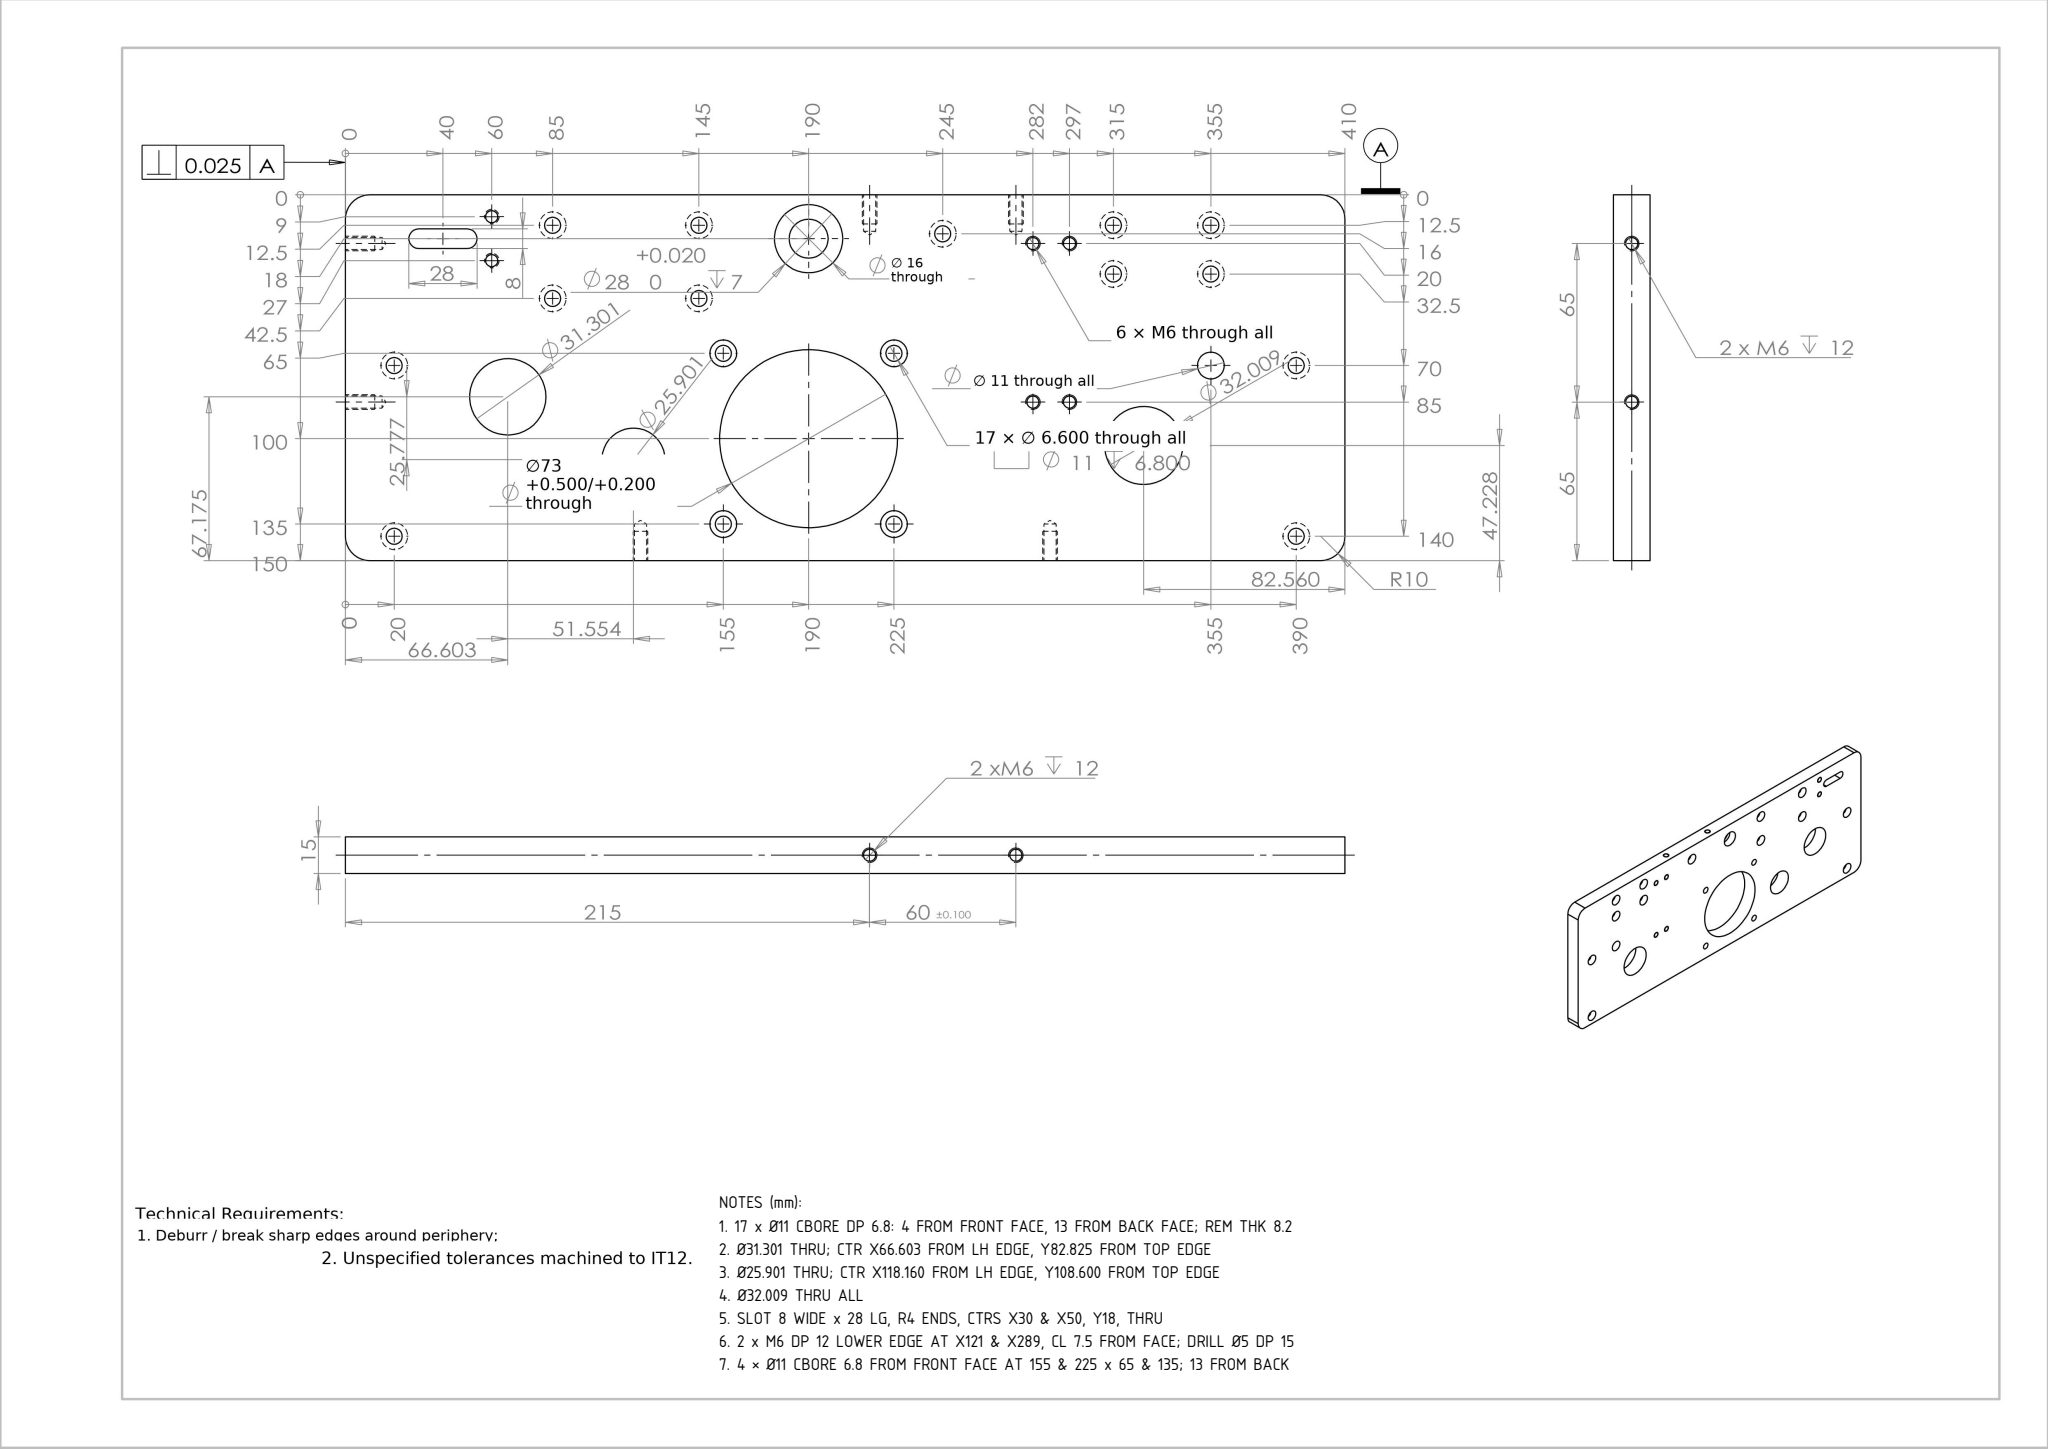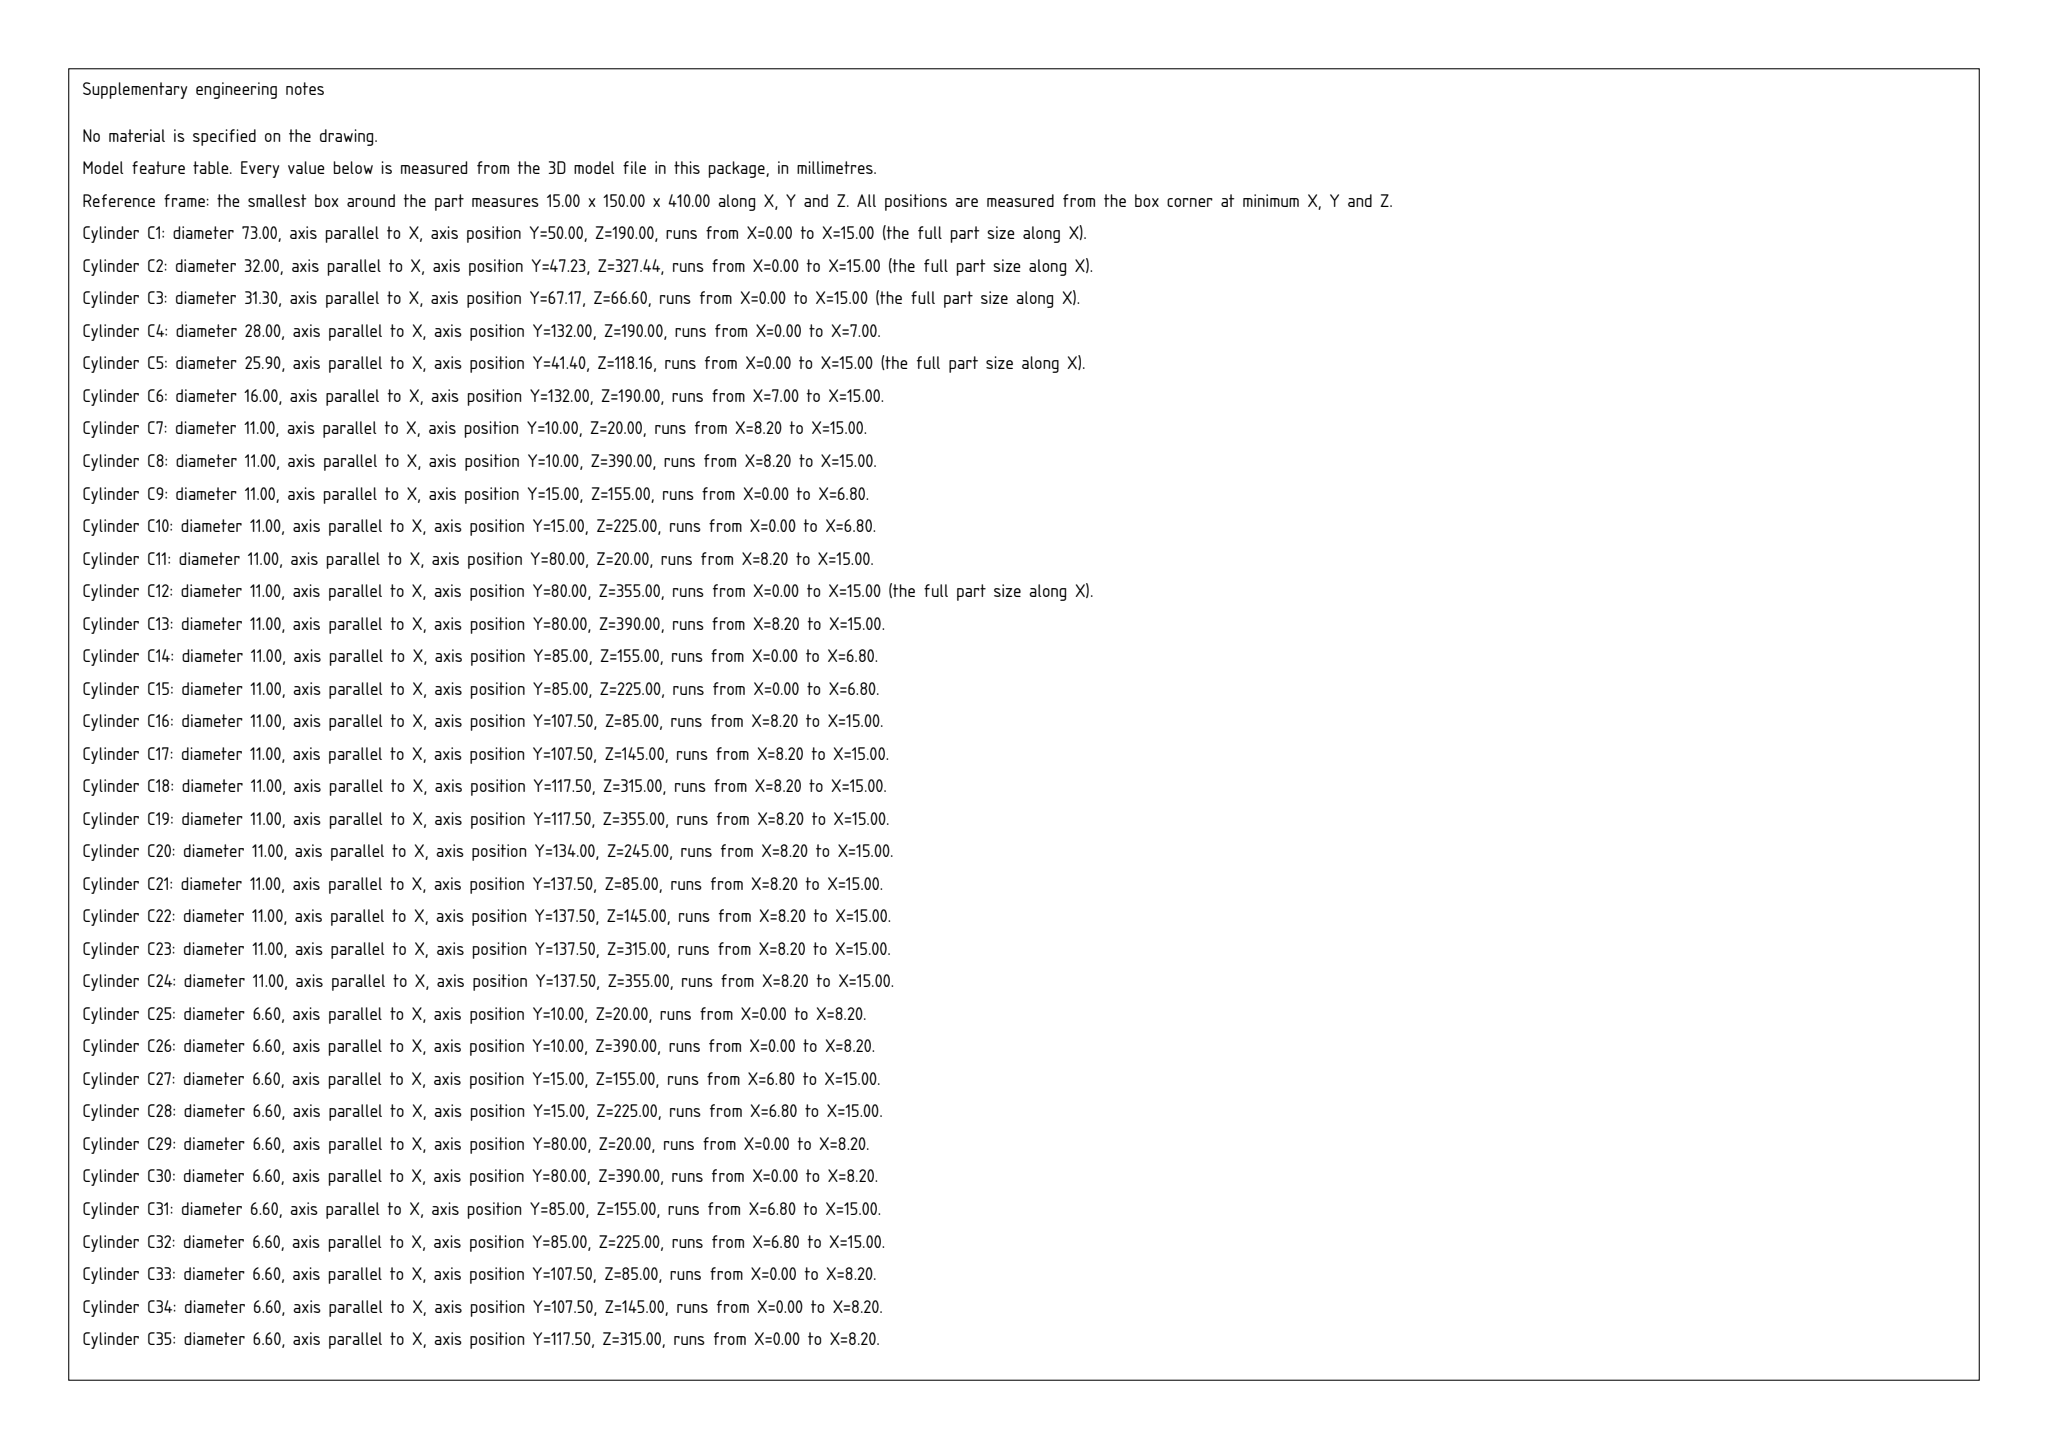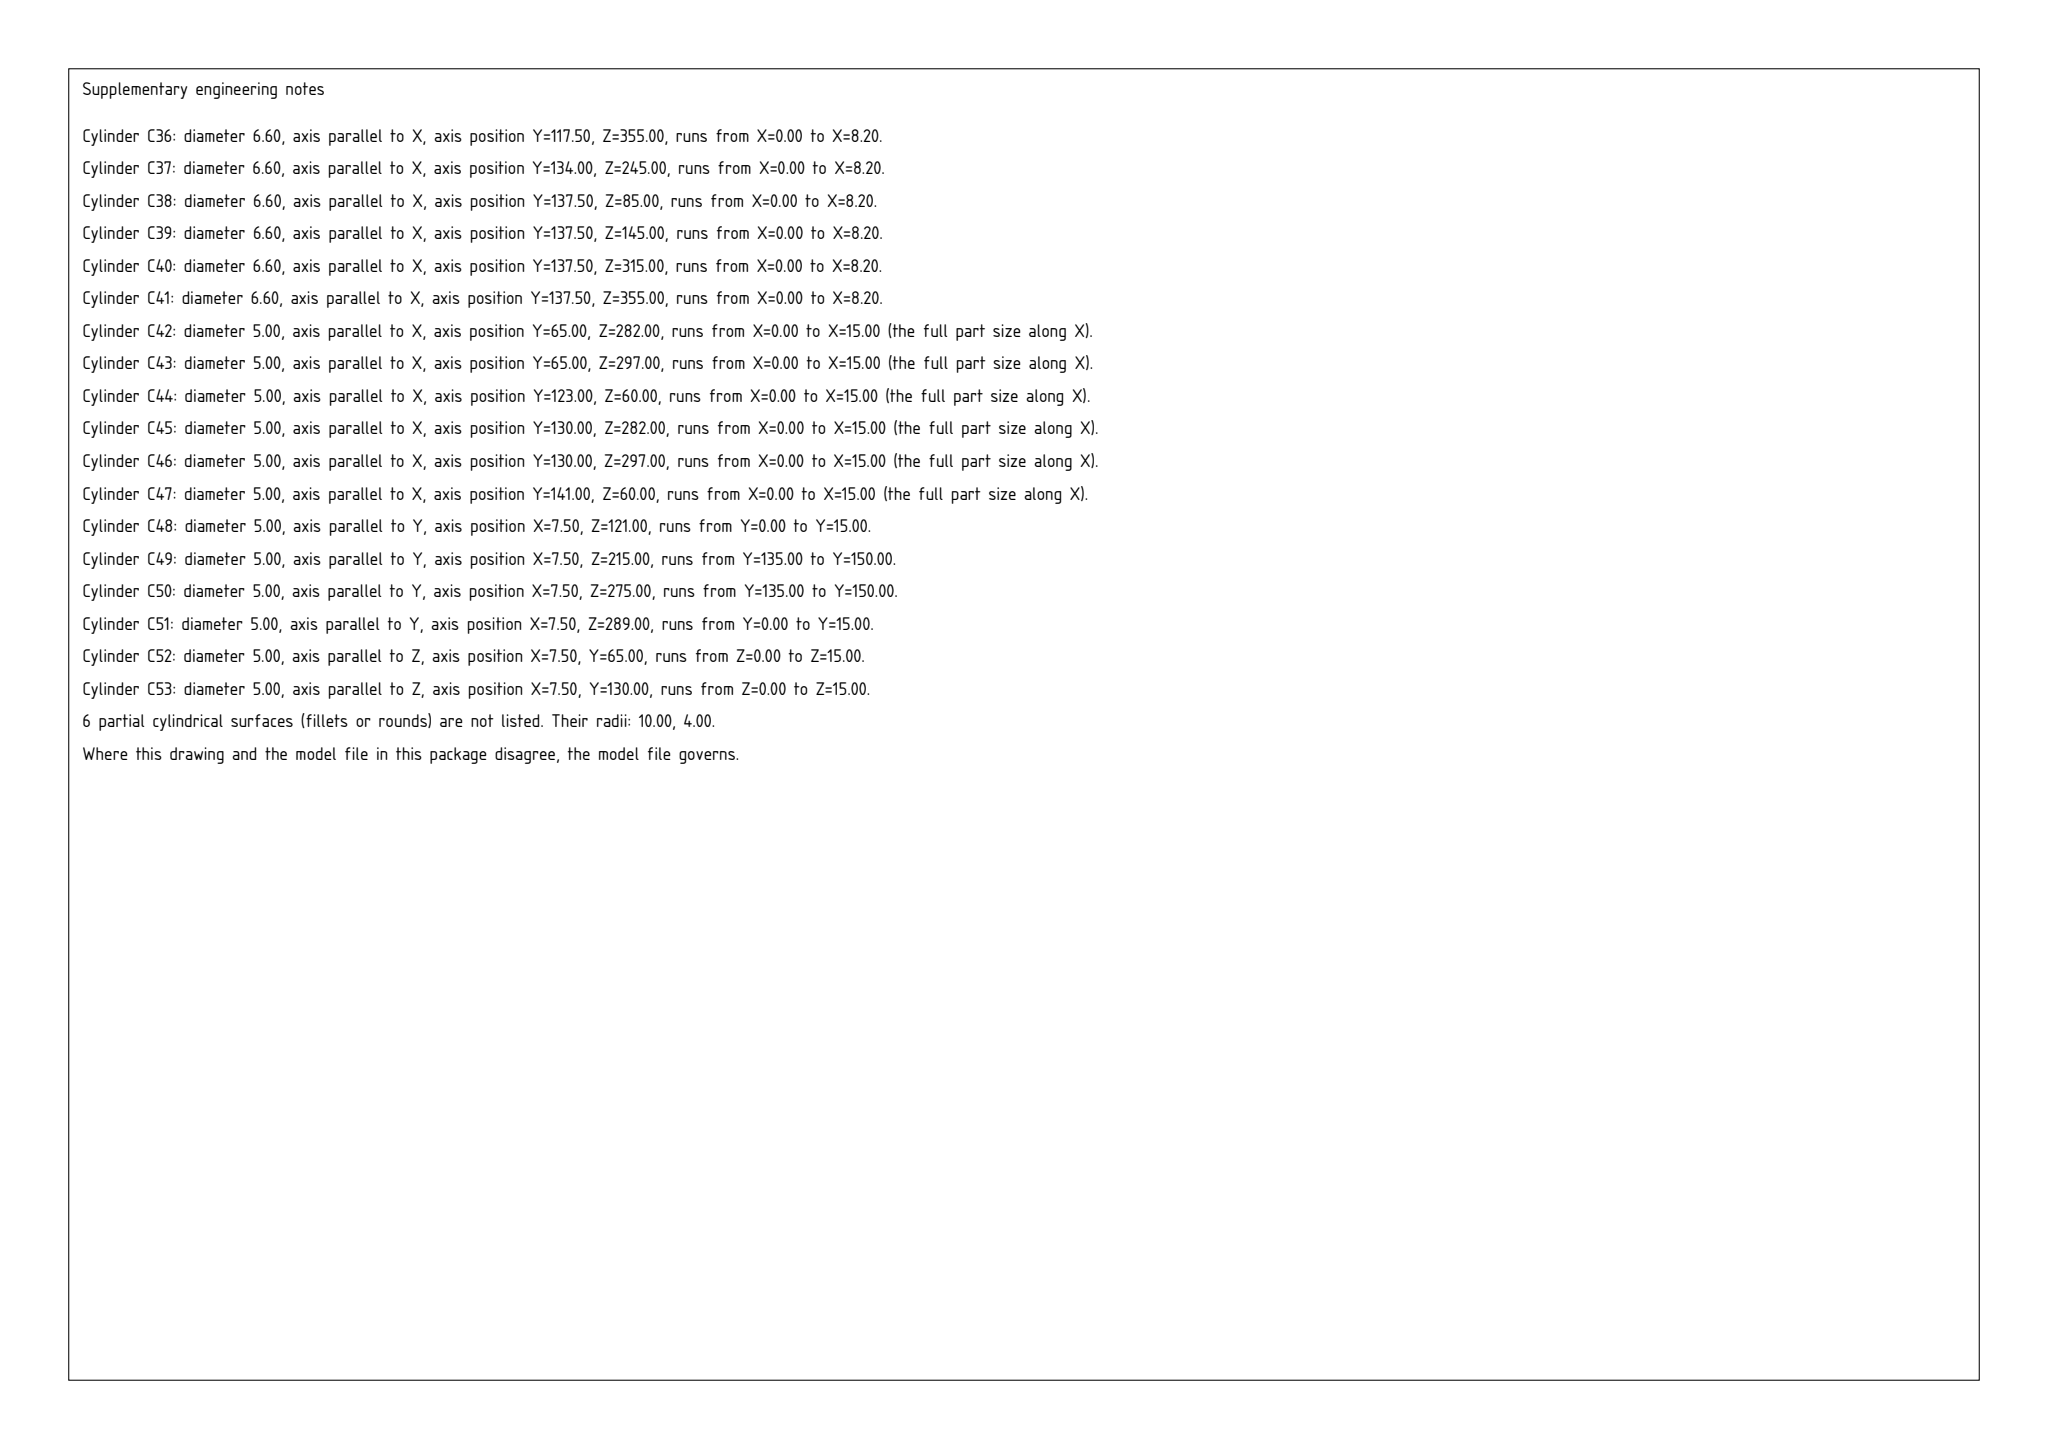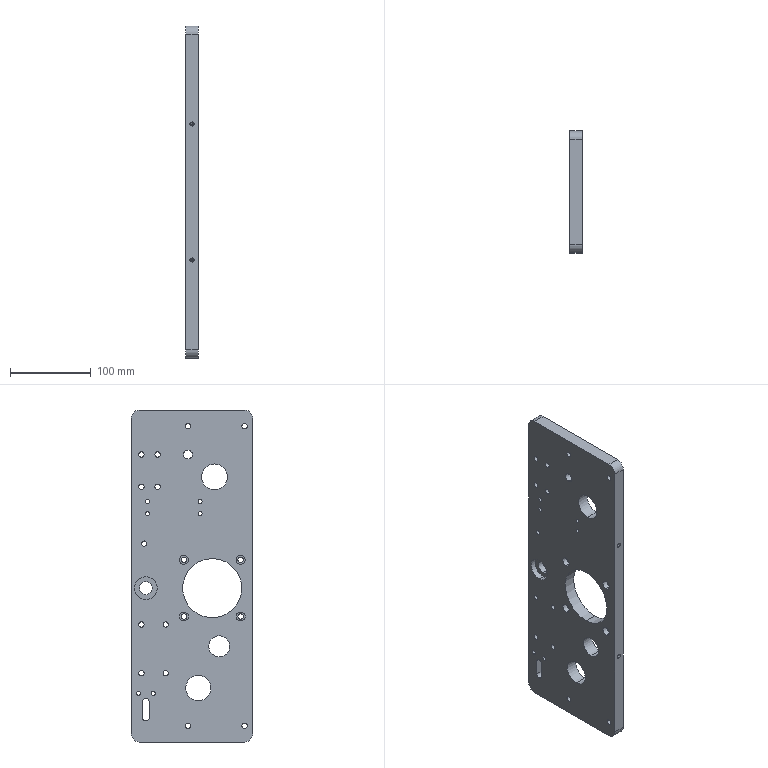Part | SolidWorks | mm | 1 solid | 151 faces | box 15 x 150 x 410 mm | volume 797070 mm3 | cylinder 113 | plane 26 | cone 12 | commonest cylinder face diameters 11 x36 6.6 x34 5 x24 20 x4 8 x3 32.009 x2 25.901 x2 31.301 x2
Drawing notes:
17 x Ø11 CBORE DP 6.8: 4 FROM FRONT FACE, 13 FROM BACK FACE; REM THK 8.2 | from the solid: axis_planes x=6.8 count 4 and x=8.2 count 13; Ø11 L6.8 x17 + Ø6.6 L8.2 x17 = 15 thk
Ø31.301 THRU; CTR X66.603 FROM LH EDGE, Y82.825 FROM TOP EDGE | from the solid: cyl Ø31.301 axis x at [y=67.17, z=66.6], L15 = plate thk; Y=150-67.175
Ø25.901 THRU; CTR X118.160 FROM LH EDGE, Y108.600 FROM TOP EDGE | from the solid: cyl Ø25.901 axis x at [y=41.4, z=118.16], L15 = plate thk; Y=150-41.4
Ø32.009 THRU ALL | from the solid: cyl Ø32.009 axis x at [y=47.23, z=327.44], L15 = plate thk
SLOT 8 WIDE x 28 LG, R4 ENDS, CTRS X30 & X50, Y18, THRU | from the solid: two Ø8 x-axis cyls at [y=132,z=30] and [y=132,z=50], L15 = thru; Y=150-132=18
2 x M6 DP 12 LOWER EDGE AT X121 & X289, CL 7.5 FROM FACE; DRILL Ø5 DP 15 | from the solid: Ø5 y-axis cyls at [x=7.5, z=121] and [x=7.5, z=289], L15; cone 118 deg ref dia 5
4 × Ø11 CBORE 6.8 FROM FRONT FACE AT 155 & 225 x 65 & 135; 13 FROM BACK | from the solid: axis_planes x=6.8 count 4 (c'bore floors opening at x=0 front face) vs x=8.2 count 13 (opening at x=15 back face); the 4 Ø11x6.8 c'bores grouped symmetric about Ø73 bore at y=15/85, z=155/225 -> 65/135 from top edge, 155/225 from left edge
build123d program:
from build123d import *

# Parameters (mm, degrees)
SKETCH1_W                                            = 360
SKETCH1_H                                            = 150
BOSS_EXTRUDE1_DEPTH                                  = 15
F_16_0_16_DIAMETER_HOLE2_D                           = 16
CUT_EXTRUDE1_DEPTH                                   = 391.288
M6_TAPPED_HOLE1_D                                    = 5
M6_TAPPED_HOLE1_DEPTH                                = 15
M6_TAPPED_HOLE1_TIP                                  = 1.502
HOLE_SIZE_ACCORDING_TO_HEX_SOCKET_HEAD_C_D           = 6.6
HOLE_SIZE_ACCORDING_TO_HEX_SOCKET_HEAD_C_CBORE_D     = 11
HOLE_SIZE_ACCORDING_TO_HEX_SOCKET_HEAD_C_CBORE_DEPTH = 6.8
HOLE_SIZE_ACCORDING_TO_HEX_SOCKET_HE_2_D             = 6.6
HOLE_SIZE_ACCORDING_TO_HEX_SOCKET_HE_2_CBORE_D       = 11
HOLE_SIZE_ACCORDING_TO_HEX_SOCKET_HE_2_CBORE_DEPTH   = 6.8
SKETCH27_R                                           = 14
CUT_EXTRUDE2_DEPTH                                   = 7
HOLE_SIZE_ACCORDING_TO_HEX_SOCKET_HE_3_D             = 6.6
HOLE_SIZE_ACCORDING_TO_HEX_SOCKET_HE_3_CBORE_D       = 11
HOLE_SIZE_ACCORDING_TO_HEX_SOCKET_HE_3_CBORE_DEPTH   = 6.8
M6_TAPPED_HOLE7_D                                    = 5
M6_TAPPED_HOLE7_DEPTH                                = 15
M6_TAPPED_HOLE7_TIP                                  = 1.502
SKETCH34_R                                           = 36.5
CUT_EXTRUDE5_DEPTH                                   = 391.288
HOLE_SIZE_ACCORDING_TO_HEX_SOCKET_HE_4_D             = 6.6
HOLE_SIZE_ACCORDING_TO_HEX_SOCKET_HE_4_CBORE_D       = 11
HOLE_SIZE_ACCORDING_TO_HEX_SOCKET_HE_4_CBORE_DEPTH   = 6.8
SKETCH39_W                                           = 15
SKETCH39_H                                           = 150
BOSS_EXTRUDE2_DEPTH                                  = 10
M6_TAPPED_HOLE6_D                                    = 5
M6_TAPPED_HOLE6_DEPTH                                = 15
M6_TAPPED_HOLE6_TIP                                  = 1.502
SKETCH40_W                                           = 15
SKETCH40_H                                           = 150
BOSS_EXTRUDE3_DEPTH                                  = 40
HOLE_SIZE_ACCORDING_TO_HEX_SOCKET_HE_5_D             = 6.6
HOLE_SIZE_ACCORDING_TO_HEX_SOCKET_HE_5_CBORE_D       = 11
HOLE_SIZE_ACCORDING_TO_HEX_SOCKET_HE_5_CBORE_DEPTH   = 6.8
M6_TAPPED_HOLE8_D                                    = 5
FILLET1_R                                            = 10
LPATTERN1_COUNT                                      = 2
LPATTERN1_PITCH                                      = 370
F_11_0_11_DIAMETER_HOLE1_D                           = 11
M6_TAPPED_HOLE9_D                                    = 5
M6_TAPPED_HOLE9_DEPTH                                = 15
M6_TAPPED_HOLE9_TIP                                  = 1.502
SKETCH49_R                                           = 16.004
SKETCH49_R_2                                         = 12.95
SKETCH49_R_3                                         = 15.65
CUT_EXTRUDE6_DEPTH                                   = 85


with BuildPart() as part:
    # Sketch1 → Boss-Extrude1 (new body)
    with BuildSketch(Plane(origin=(0, 0, 0), x_dir=(0, 0, -1), z_dir=(1, 0, 0))):
        with Locations((180, 75)):
            Rectangle(SKETCH1_W, SKETCH1_H)
    extrude(amount=BOSS_EXTRUDE1_DEPTH)

    # 16.0 _16_ Diameter Hole2 (through all)
    with Locations(Plane(origin=(15, 0, 0), x_dir=(0, 0, -1), z_dir=(1, 0, 0))):
        with Locations((180, 132)):
            Hole(F_16_0_16_DIAMETER_HOLE2_D / 2)

    # Sketch8 → Cut-Extrude1 (cut, through all)
    with BuildSketch(Plane(origin=(15, 0, 0), x_dir=(0, 0, -1), z_dir=(1, 0, 0))):
        with BuildLine():
            Line((320, 136), (340, 136))
            ThreePointArc((340, 136), (344, 132), (340, 128))
            Line((340, 128), (320, 128))
            ThreePointArc((320, 128), (316, 132), (320, 136))
        make_face()
    extrude(amount=-CUT_EXTRUDE1_DEPTH, mode=Mode.SUBTRACT)

    # M6 Tapped Hole1
    with Locations(Plane(origin=(15, 0, 0), x_dir=(0, 0, -1), z_dir=(1, 0, 0))):
        with Locations((310, 141), (310, 123)):
            Hole(M6_TAPPED_HOLE1_D / 2, depth=M6_TAPPED_HOLE1_DEPTH)
            with Locations((0, 0, -(M6_TAPPED_HOLE1_DEPTH + M6_TAPPED_HOLE1_TIP / 2))):  # 118° drill point
                Cone(0, M6_TAPPED_HOLE1_D / 2, M6_TAPPED_HOLE1_TIP, mode=Mode.SUBTRACT)

    # Hole Size according to Hex Socket Head C (through all)
    with Locations(Plane(origin=(15, 0, 0), x_dir=(0, 0, -1), z_dir=(1, 0, 0))):
        with Locations((350, 10), (350, 80)):
            hole_size_according_to_hex_socket_head_c = CounterBoreHole(HOLE_SIZE_ACCORDING_TO_HEX_SOCKET_HEAD_C_D / 2, HOLE_SIZE_ACCORDING_TO_HEX_SOCKET_HEAD_C_CBORE_D / 2, HOLE_SIZE_ACCORDING_TO_HEX_SOCKET_HEAD_C_CBORE_DEPTH)

    # Hole Size according to Hex Socket He 2 (through all)
    with Locations(Plane(origin=(15, 0, 0), x_dir=(0, 0, -1), z_dir=(1, 0, 0))):
        with Locations((285, 107.5), (225, 107.5), (285, 137.5), (225, 137.5)):
            CounterBoreHole(HOLE_SIZE_ACCORDING_TO_HEX_SOCKET_HE_2_D / 2, HOLE_SIZE_ACCORDING_TO_HEX_SOCKET_HE_2_CBORE_D / 2, HOLE_SIZE_ACCORDING_TO_HEX_SOCKET_HE_2_CBORE_DEPTH)

    # Sketch27 → Cut-Extrude2 (cut)
    with BuildSketch(Plane.ZY):
        with Locations((-180, 132)):
            Circle(SKETCH27_R)
    extrude(amount=-CUT_EXTRUDE2_DEPTH, mode=Mode.SUBTRACT)

    # Hole Size according to Hex Socket He 3 (through all)
    with Locations(Plane(origin=(15, 0, 0), x_dir=(0, 0, -1), z_dir=(1, 0, 0))):
        with Locations((125, 134)):
            CounterBoreHole(HOLE_SIZE_ACCORDING_TO_HEX_SOCKET_HE_3_D / 2, HOLE_SIZE_ACCORDING_TO_HEX_SOCKET_HE_3_CBORE_D / 2, HOLE_SIZE_ACCORDING_TO_HEX_SOCKET_HE_3_CBORE_DEPTH)

    # M6 Tapped Hole7
    with Locations(Plane(origin=(0, 150, 0), x_dir=(-1, 0, 0), z_dir=(0, 1, 0))):
        with Locations((-7.5, -155), (-7.5, -95)):
            Hole(M6_TAPPED_HOLE7_D / 2, depth=M6_TAPPED_HOLE7_DEPTH)
            with Locations((0, 0, -(M6_TAPPED_HOLE7_DEPTH + M6_TAPPED_HOLE7_TIP / 2))):  # 118° drill point
                Cone(0, M6_TAPPED_HOLE7_D / 2, M6_TAPPED_HOLE7_TIP, mode=Mode.SUBTRACT)

    # Sketch34 → Cut-Extrude5 (cut, through all)
    with BuildSketch(Plane.ZY):
        with Locations((-180, 50)):
            Circle(SKETCH34_R)
    extrude(amount=-CUT_EXTRUDE5_DEPTH, mode=Mode.SUBTRACT)

    # Hole Size according to Hex Socket He 4 (through all)
    with Locations(Plane.ZY):
        with Locations((-215, 85), (-145, 85), (-145, 15), (-215, 15)):
            CounterBoreHole(HOLE_SIZE_ACCORDING_TO_HEX_SOCKET_HE_4_D / 2, HOLE_SIZE_ACCORDING_TO_HEX_SOCKET_HE_4_CBORE_D / 2, HOLE_SIZE_ACCORDING_TO_HEX_SOCKET_HE_4_CBORE_DEPTH)

    # Sketch39 → Boss-Extrude2 (add)
    with BuildSketch(Plane(origin=(0, 0, -360), x_dir=(-1, 0, 0), z_dir=(0, 0, -1))):
        with Locations((-7.5, 75)):
            Rectangle(SKETCH39_W, SKETCH39_H)
    extrude(amount=BOSS_EXTRUDE2_DEPTH)

    # M6 Tapped Hole6
    with Locations(Plane(origin=(0.007088, 11.918, -370), x_dir=(-1, 0, 0), z_dir=(0, 0, -1))):
        with Locations((-7.493, 118.082), (-7.493, 53.082)):
            Hole(M6_TAPPED_HOLE6_D / 2, depth=M6_TAPPED_HOLE6_DEPTH)
            with Locations((0, 0, -(M6_TAPPED_HOLE6_DEPTH + M6_TAPPED_HOLE6_TIP / 2))):  # 118° drill point
                Cone(0, M6_TAPPED_HOLE6_D / 2, M6_TAPPED_HOLE6_TIP, mode=Mode.SUBTRACT)

    # Sketch40 → Boss-Extrude3 (add)
    with BuildSketch(Plane.XY):
        with Locations((7.5, 75)):
            Rectangle(SKETCH40_W, SKETCH40_H)
    extrude(amount=BOSS_EXTRUDE3_DEPTH)

    # Hole Size according to Hex Socket He 5 (through all)
    with Locations(Plane(origin=(15, 0, 0), x_dir=(0, 0, -1), z_dir=(1, 0, 0))):
        with Locations((15, 137.5), (55, 137.5), (55, 117.5), (15, 117.5)):
            CounterBoreHole(HOLE_SIZE_ACCORDING_TO_HEX_SOCKET_HE_5_D / 2, HOLE_SIZE_ACCORDING_TO_HEX_SOCKET_HE_5_CBORE_D / 2, HOLE_SIZE_ACCORDING_TO_HEX_SOCKET_HE_5_CBORE_DEPTH)

    # M6 Tapped Hole8 (through all)
    with Locations(Plane(origin=(15, 0, 0), x_dir=(0, 0, -1), z_dir=(1, 0, 0))):
        with Locations((73, 65), (73, 130), (88, 130), (88, 65)):
            Hole(M6_TAPPED_HOLE8_D / 2)

    # Fillet1
    fillet1_edges = [part.edges().sort_by_distance(p)[0] for p in [
        (7.5, 0, -370),
        (7.5, 150, -370),
        (7.5, 0, 40),
        (7.5, 150, 40),
    ]]
    fillet(fillet1_edges, radius=FILLET1_R)

    # LPattern1: Hole Size according to Hex Socket Head C ×2
    with Locations(*[(0, 0, i * LPATTERN1_PITCH) for i in range(1, LPATTERN1_COUNT)]):
        add(hole_size_according_to_hex_socket_head_c, mode=Mode.SUBTRACT)

    # 11.0 _11_ Diameter Hole1 (through all)
    with Locations(Plane(origin=(15, 0, 0), x_dir=(0, 0, -1), z_dir=(1, 0, 0))):
        with Locations((15, 80)):
            Hole(F_11_0_11_DIAMETER_HOLE1_D / 2)

    # M6 Tapped Hole9
    with Locations(Plane.XZ):
        with Locations((7.5, -81), (7.5, -249)):
            Hole(M6_TAPPED_HOLE9_D / 2, depth=M6_TAPPED_HOLE9_DEPTH)
            with Locations((0, 0, -(M6_TAPPED_HOLE9_DEPTH + M6_TAPPED_HOLE9_TIP / 2))):  # 118° drill point
                Cone(0, M6_TAPPED_HOLE9_D / 2, M6_TAPPED_HOLE9_TIP, mode=Mode.SUBTRACT)

    # Sketch49 → Cut-Extrude6 (cut)
    with BuildSketch(Plane(origin=(15, 0, 0), x_dir=(0, 0, -1), z_dir=(1, 0, 0))):
        with Locations((42.56, 47.228)):
            Circle(SKETCH49_R)
        with Locations((251.844, 41.398)):
            Circle(SKETCH49_R_2)
        with Locations((303.397, 67.175)):
            Circle(SKETCH49_R_3)
    extrude(amount=-CUT_EXTRUDE6_DEPTH, mode=Mode.SUBTRACT)


solid = part.part